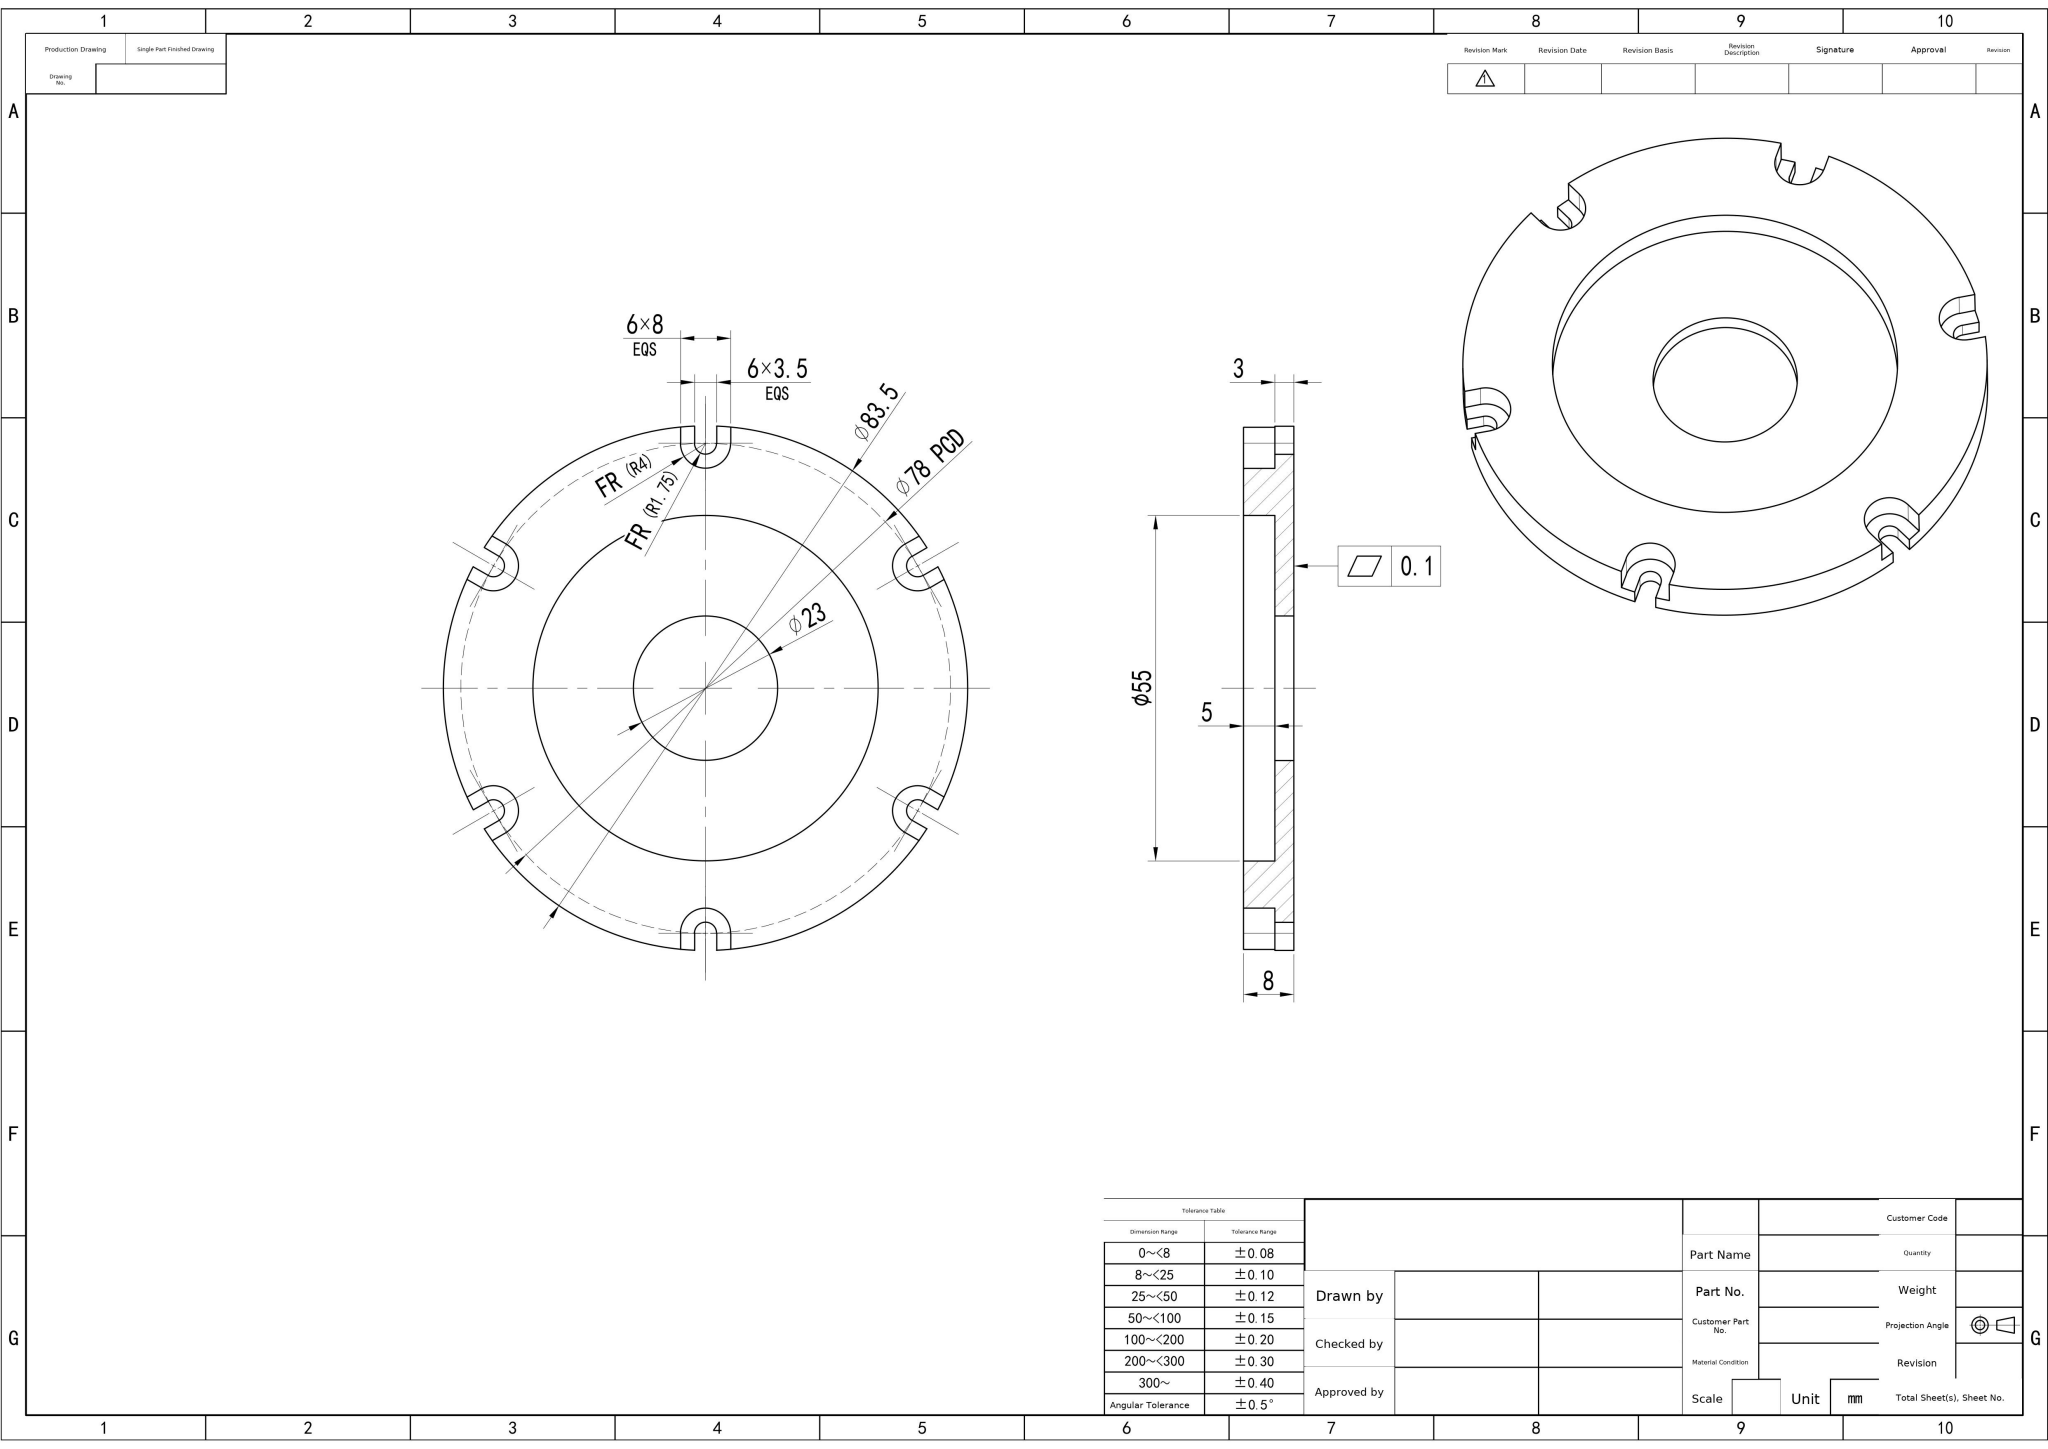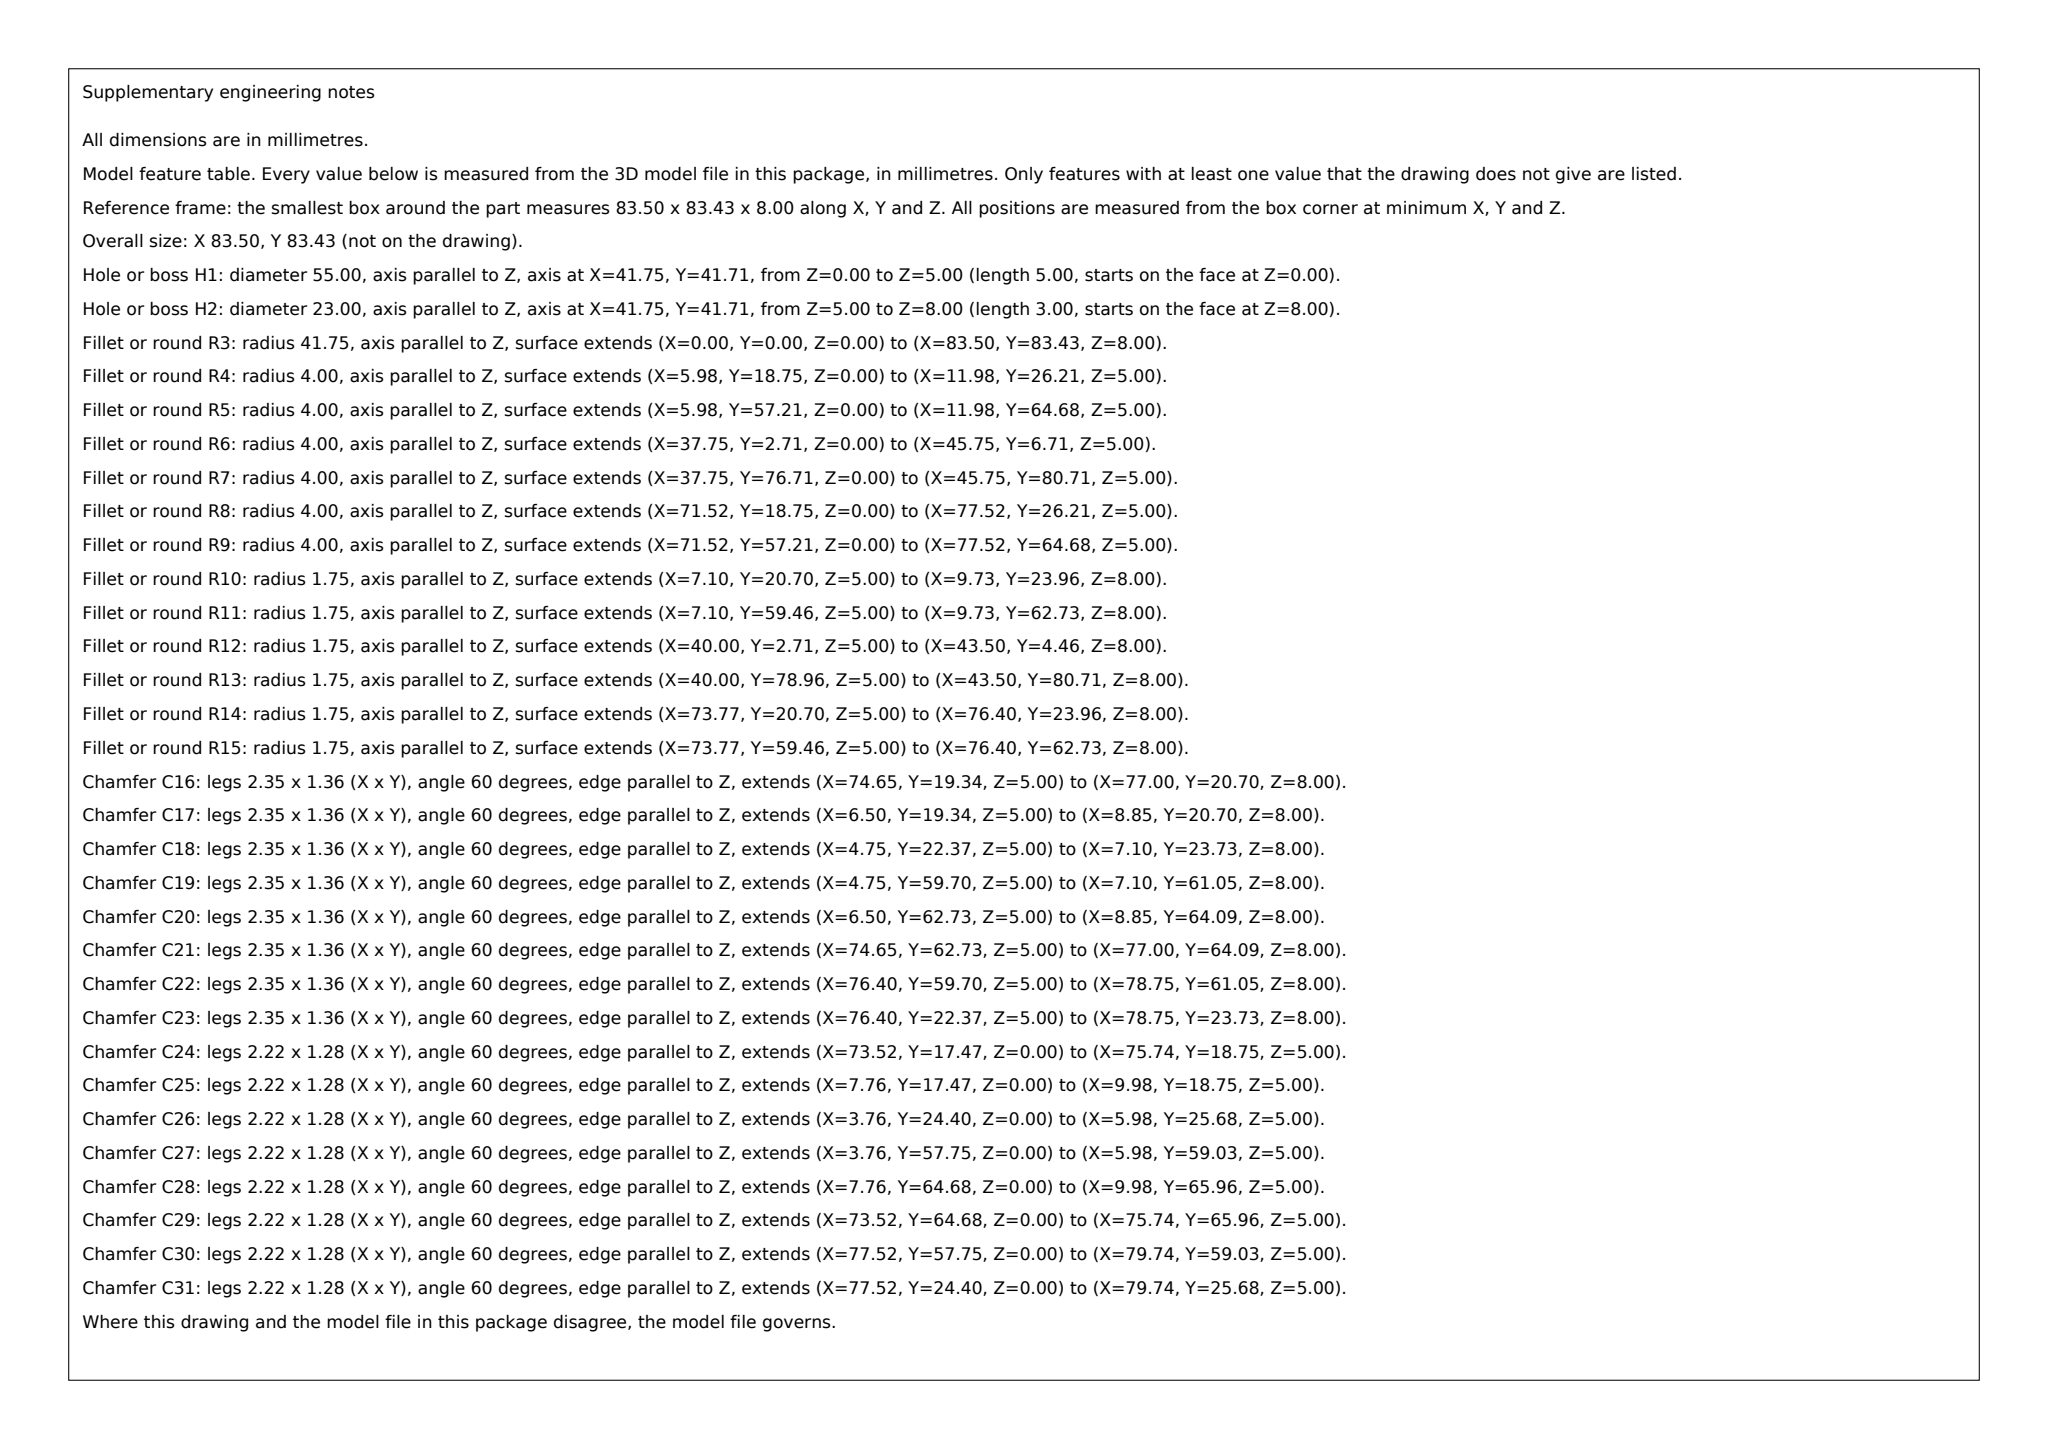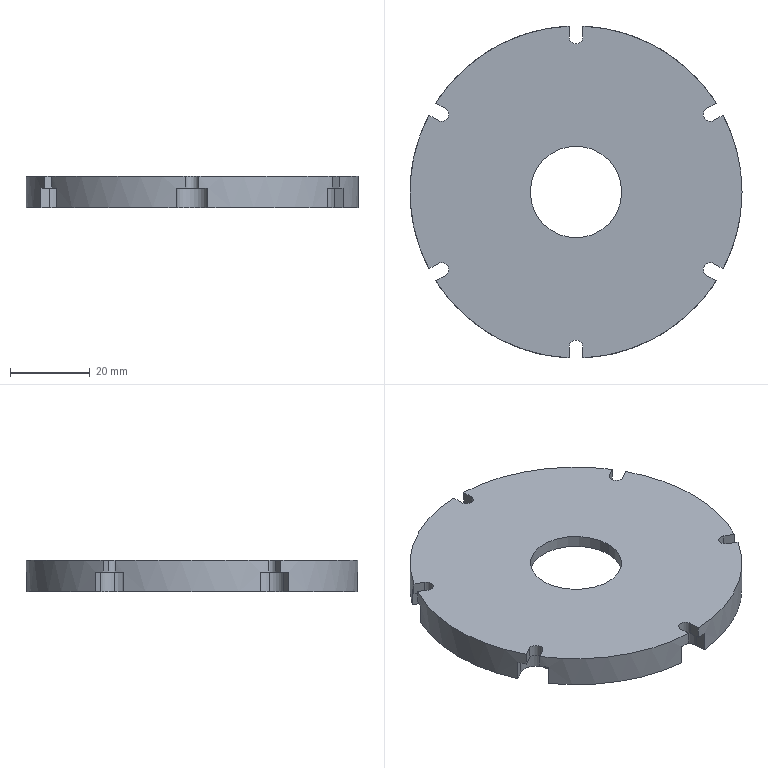Part | SolidWorks | mm | 1 solid | 60 faces | box 83.5 x 83.43 x 8 mm | volume 29025 mm3 | plane 33 | cylinder 27 | commonest cylinder face diameters 3.5 x8 8 x8 83.5 x7 23 x2 55 x2